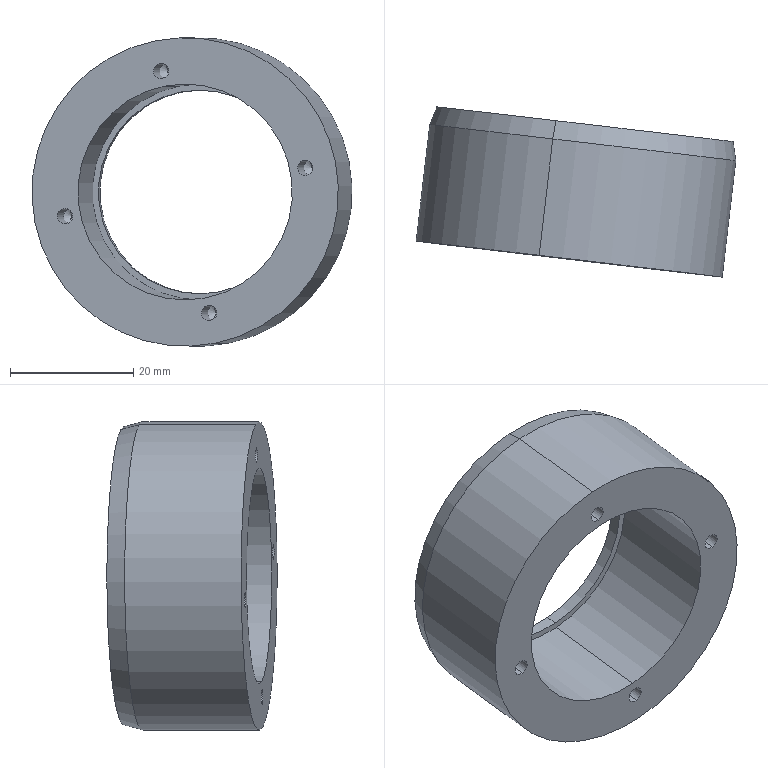Component | SolidWorks | 8TC-A17001-91-00UpperAndLowerPressAssembly-1_8TC-A17001-91-04PressureRoller-1 | 1 solid | 27 faces | box 51.88 x 27.59 x 50 mm | volume 21885 mm3 | cylinder 14 | cone 10 | plane 3 | commonest cylinder face diameters 2.5 x8 33 x2 50 x2 35 x2 | material Cr12MoV
STEP:
#1=COLOUR_RGB('',0.7922,0.8196,0.9333);
#2=FILL_AREA_STYLE_COLOUR('',#1);
#3=FILL_AREA_STYLE('',(#2));
#4=SURFACE_STYLE_FILL_AREA(#3);
#5=SURFACE_SIDE_STYLE('',(#4));
#6=SURFACE_STYLE_USAGE(.BOTH.,#5);
#7=PRESENTATION_STYLE_ASSIGNMENT((#6));
#8=CARTESIAN_POINT('',(0.232,-2.897,-2.771));
#9=VERTEX_POINT('',#8);
#10=CARTESIAN_POINT('',(0.2512,-2.899,-2.868));
#11=VERTEX_POINT('',#10);
#12=CARTESIAN_POINT('',(0.2416,-2.898,-2.819));
#13=DIRECTION('',(-0.1167,-0.9932,0.));
#14=DIRECTION('',(0.1946,-0.02286,-0.9806));
#15=AXIS2_PLACEMENT_3D('',#12,#13,#14);
#16=CIRCLE('',#15,0.04921);
#17=EDGE_CURVE('',#9,#11,#16,.T.);
#18=ORIENTED_EDGE('',*,*,#17,.F.);
#19=CARTESIAN_POINT('',(0.193,-3.229,-2.771));
#20=VERTEX_POINT('',#19);
#21=CARTESIAN_POINT('',(0.193,-3.229,-2.771));
#22=DIRECTION('',(-0.1167,-0.9932,0.));
#23=VECTOR('',#22,39.37);
#24=LINE('',#21,#23);
#25=EDGE_CURVE('',#9,#20,#24,.T.);
#26=ORIENTED_EDGE('',*,*,#25,.T.);
#27=CARTESIAN_POINT('',(0.2122,-3.231,-2.868));
#28=VERTEX_POINT('',#27);
#29=CARTESIAN_POINT('',(0.2026,-3.23,-2.819));
#30=DIRECTION('',(-0.1167,-0.9932,0.));
#31=DIRECTION('',(0.1946,-0.02286,-0.9806));
#32=AXIS2_PLACEMENT_3D('',#29,#30,#31);
#33=CIRCLE('',#32,0.04921);
#34=EDGE_CURVE('',#20,#28,#33,.T.);
#35=ORIENTED_EDGE('',*,*,#34,.T.);
#36=CARTESIAN_POINT('',(0.2122,-3.231,-2.868));
#37=DIRECTION('',(-0.1167,-0.9932,0.));
#38=VECTOR('',#37,39.37);
#39=LINE('',#36,#38);
#40=EDGE_CURVE('',#11,#28,#39,.T.);
#41=ORIENTED_EDGE('',*,*,#40,.F.);
#42=EDGE_LOOP('',(#18,#26,#35,#41));
#43=FACE_OUTER_BOUND('',#42,.T.);
#44=CARTESIAN_POINT('',(0.2026,-3.23,-2.819));
#45=DIRECTION('',(-0.1167,-0.9932,0.));
#46=DIRECTION('',(0.1946,-0.02286,-0.9806));
#47=AXIS2_PLACEMENT_3D('',#44,#45,#46);
#48=CYLINDRICAL_SURFACE('',#47,0.04921);
#49=ADVANCED_FACE('',(#43),#48,.F.);
#50=CARTESIAN_POINT('',(0.2451,-2.868,-2.819));
#51=VERTEX_POINT('',#50);
#52=CARTESIAN_POINT('',(0.2512,-2.899,-2.868));
#53=DIRECTION('',(0.1067,-0.5311,-0.8406));
#54=VECTOR('',#53,39.37);
#55=LINE('',#52,#54);
#56=EDGE_CURVE('',#51,#11,#55,.T.);
#57=ORIENTED_EDGE('',*,*,#56,.F.);
#58=CARTESIAN_POINT('',(0.232,-2.897,-2.771));
#59=DIRECTION('',(-0.2269,-0.4919,0.8406));
#60=VECTOR('',#59,39.37);
#61=LINE('',#58,#60);
#62=EDGE_CURVE('',#51,#9,#61,.T.);
#63=ORIENTED_EDGE('',*,*,#62,.T.);
#64=ORIENTED_EDGE('',*,*,#17,.T.);
#65=EDGE_LOOP('',(#57,#63,#64));
#66=FACE_OUTER_BOUND('',#65,.T.);
#67=CARTESIAN_POINT('',(0.2416,-2.898,-2.819));
#68=DIRECTION('',(-0.1167,-0.9932,0.));
#69=DIRECTION('',(0.1946,-0.02286,-0.9806));
#70=AXIS2_PLACEMENT_3D('',#67,#68,#69);
#71=CONICAL_SURFACE('',#70,0.04921,1.03);
#72=ADVANCED_FACE('',(#66),#71,.F.);
#73=CARTESIAN_POINT('',(0.8457,-2.969,-1.845));
#74=VERTEX_POINT('',#73);
#75=CARTESIAN_POINT('',(0.8648,-2.971,-1.941));
#76=VERTEX_POINT('',#75);
#77=CARTESIAN_POINT('',(0.8553,-2.97,-1.893));
#78=DIRECTION('',(-0.1167,-0.9932,0.));
#79=DIRECTION('',(0.1946,-0.02286,-0.9806));
#80=AXIS2_PLACEMENT_3D('',#77,#78,#79);
#81=CIRCLE('',#80,0.04921);
#82=EDGE_CURVE('',#74,#76,#81,.T.);
#83=ORIENTED_EDGE('',*,*,#82,.F.);
#84=CARTESIAN_POINT('',(0.8066,-3.301,-1.845));
#85=VERTEX_POINT('',#84);
#86=CARTESIAN_POINT('',(0.8066,-3.301,-1.845));
#87=DIRECTION('',(-0.1167,-0.9932,0.));
#88=VECTOR('',#87,39.37);
#89=LINE('',#86,#88);
#90=EDGE_CURVE('',#74,#85,#89,.T.);
#91=ORIENTED_EDGE('',*,*,#90,.T.);
#92=CARTESIAN_POINT('',(0.8258,-3.303,-1.941));
#93=VERTEX_POINT('',#92);
#94=CARTESIAN_POINT('',(0.8162,-3.302,-1.893));
#95=DIRECTION('',(-0.1167,-0.9932,0.));
#96=DIRECTION('',(0.1946,-0.02286,-0.9806));
#97=AXIS2_PLACEMENT_3D('',#94,#95,#96);
#98=CIRCLE('',#97,0.04921);
#99=EDGE_CURVE('',#85,#93,#98,.T.);
#100=ORIENTED_EDGE('',*,*,#99,.T.);
#101=CARTESIAN_POINT('',(0.8258,-3.303,-1.941));
#102=DIRECTION('',(-0.1167,-0.9932,0.));
#103=VECTOR('',#102,39.37);
#104=LINE('',#101,#103);
#105=EDGE_CURVE('',#76,#93,#104,.T.);
#106=ORIENTED_EDGE('',*,*,#105,.F.);
#107=EDGE_LOOP('',(#83,#91,#100,#106));
#108=FACE_OUTER_BOUND('',#107,.T.);
#109=CARTESIAN_POINT('',(0.8162,-3.302,-1.893));
#110=DIRECTION('',(-0.1167,-0.9932,0.));
#111=DIRECTION('',(0.1946,-0.02286,-0.9806));
#112=AXIS2_PLACEMENT_3D('',#109,#110,#111);
#113=CYLINDRICAL_SURFACE('',#112,0.04921);
#114=ADVANCED_FACE('',(#108),#113,.F.);
#115=CARTESIAN_POINT('',(0.8587,-2.94,-1.893));
#116=VERTEX_POINT('',#115);
#117=CARTESIAN_POINT('',(0.8648,-2.971,-1.941));
#118=DIRECTION('',(0.1067,-0.5311,-0.8406));
#119=VECTOR('',#118,39.37);
#120=LINE('',#117,#119);
#121=EDGE_CURVE('',#116,#76,#120,.T.);
#122=ORIENTED_EDGE('',*,*,#121,.F.);
#123=CARTESIAN_POINT('',(0.8457,-2.969,-1.845));
#124=DIRECTION('',(-0.2269,-0.4919,0.8406));
#125=VECTOR('',#124,39.37);
#126=LINE('',#123,#125);
#127=EDGE_CURVE('',#116,#74,#126,.T.);
#128=ORIENTED_EDGE('',*,*,#127,.T.);
#129=ORIENTED_EDGE('',*,*,#82,.T.);
#130=EDGE_LOOP('',(#122,#128,#129));
#131=FACE_OUTER_BOUND('',#130,.T.);
#132=CARTESIAN_POINT('',(0.8553,-2.97,-1.893));
#133=DIRECTION('',(-0.1167,-0.9932,0.));
#134=DIRECTION('',(0.1946,-0.02286,-0.9806));
#135=AXIS2_PLACEMENT_3D('',#132,#133,#134);
#136=CONICAL_SURFACE('',#135,0.04921,1.03);
#137=ADVANCED_FACE('',(#131),#136,.F.);
#138=CARTESIAN_POINT('',(-0.07442,-2.861,-1.227));
#139=VERTEX_POINT('',#138);
#140=CARTESIAN_POINT('',(-0.05527,-2.863,-1.323));
#141=VERTEX_POINT('',#140);
#142=CARTESIAN_POINT('',(-0.06484,-2.862,-1.275));
#143=DIRECTION('',(-0.1167,-0.9932,0.));
#144=DIRECTION('',(0.1946,-0.02286,-0.9806));
#145=AXIS2_PLACEMENT_3D('',#142,#143,#144);
#146=CIRCLE('',#145,0.04921);
#147=EDGE_CURVE('',#139,#141,#146,.T.);
#148=ORIENTED_EDGE('',*,*,#147,.F.);
#149=CARTESIAN_POINT('',(-0.1135,-3.193,-1.227));
#150=VERTEX_POINT('',#149);
#151=CARTESIAN_POINT('',(-0.1135,-3.193,-1.227));
#152=DIRECTION('',(-0.1167,-0.9932,0.));
#153=VECTOR('',#152,39.37);
#154=LINE('',#151,#153);
#155=EDGE_CURVE('',#139,#150,#154,.T.);
#156=ORIENTED_EDGE('',*,*,#155,.T.);
#157=CARTESIAN_POINT('',(-0.09431,-3.195,-1.323));
#158=VERTEX_POINT('',#157);
#159=CARTESIAN_POINT('',(-0.1039,-3.194,-1.275));
#160=DIRECTION('',(-0.1167,-0.9932,0.));
#161=DIRECTION('',(0.1946,-0.02286,-0.9806));
#162=AXIS2_PLACEMENT_3D('',#159,#160,#161);
#163=CIRCLE('',#162,0.04921);
#164=EDGE_CURVE('',#150,#158,#163,.T.);
#165=ORIENTED_EDGE('',*,*,#164,.T.);
#166=CARTESIAN_POINT('',(-0.09431,-3.195,-1.323));
#167=DIRECTION('',(-0.1167,-0.9932,0.));
#168=VECTOR('',#167,39.37);
#169=LINE('',#166,#168);
#170=EDGE_CURVE('',#141,#158,#169,.T.);
#171=ORIENTED_EDGE('',*,*,#170,.F.);
#172=EDGE_LOOP('',(#148,#156,#165,#171));
#173=FACE_OUTER_BOUND('',#172,.T.);
#174=CARTESIAN_POINT('',(-0.1039,-3.194,-1.275));
#175=DIRECTION('',(-0.1167,-0.9932,0.));
#176=DIRECTION('',(0.1946,-0.02286,-0.9806));
#177=AXIS2_PLACEMENT_3D('',#174,#175,#176);
#178=CYLINDRICAL_SURFACE('',#177,0.04921);
#179=ADVANCED_FACE('',(#173),#178,.F.);
#180=CARTESIAN_POINT('',(-0.0614,-2.832,-1.275));
#181=VERTEX_POINT('',#180);
#182=CARTESIAN_POINT('',(-0.05527,-2.863,-1.323));
#183=DIRECTION('',(0.1067,-0.5311,-0.8406));
#184=VECTOR('',#183,39.37);
#185=LINE('',#182,#184);
#186=EDGE_CURVE('',#181,#141,#185,.T.);
#187=ORIENTED_EDGE('',*,*,#186,.F.);
#188=CARTESIAN_POINT('',(-0.07442,-2.861,-1.227));
#189=DIRECTION('',(-0.2269,-0.4919,0.8406));
#190=VECTOR('',#189,39.37);
#191=LINE('',#188,#190);
#192=EDGE_CURVE('',#181,#139,#191,.T.);
#193=ORIENTED_EDGE('',*,*,#192,.T.);
#194=ORIENTED_EDGE('',*,*,#147,.T.);
#195=EDGE_LOOP('',(#187,#193,#194));
#196=FACE_OUTER_BOUND('',#195,.T.);
#197=CARTESIAN_POINT('',(-0.06484,-2.862,-1.275));
#198=DIRECTION('',(-0.1167,-0.9932,0.));
#199=DIRECTION('',(0.1946,-0.02286,-0.9806));
#200=AXIS2_PLACEMENT_3D('',#197,#198,#199);
#201=CONICAL_SURFACE('',#200,0.04921,1.03);
#202=ADVANCED_FACE('',(#196),#201,.F.);
#203=CARTESIAN_POINT('',(-0.6881,-2.788,-2.153));
#204=VERTEX_POINT('',#203);
#205=CARTESIAN_POINT('',(-0.6689,-2.791,-2.25));
#206=VERTEX_POINT('',#205);
#207=CARTESIAN_POINT('',(-0.6785,-2.79,-2.202));
#208=DIRECTION('',(-0.1167,-0.9932,0.));
#209=DIRECTION('',(0.1946,-0.02286,-0.9806));
#210=AXIS2_PLACEMENT_3D('',#207,#208,#209);
#211=CIRCLE('',#210,0.04921);
#212=EDGE_CURVE('',#204,#206,#211,.T.);
#213=ORIENTED_EDGE('',*,*,#212,.F.);
#214=CARTESIAN_POINT('',(-0.7271,-3.121,-2.153));
#215=VERTEX_POINT('',#214);
#216=CARTESIAN_POINT('',(-0.7271,-3.121,-2.153));
#217=DIRECTION('',(-0.1167,-0.9932,0.));
#218=VECTOR('',#217,39.37);
#219=LINE('',#216,#218);
#220=EDGE_CURVE('',#204,#215,#219,.T.);
#221=ORIENTED_EDGE('',*,*,#220,.T.);
#222=CARTESIAN_POINT('',(-0.7079,-3.123,-2.25));
#223=VERTEX_POINT('',#222);
#224=CARTESIAN_POINT('',(-0.7175,-3.122,-2.202));
#225=DIRECTION('',(-0.1167,-0.9932,0.));
#226=DIRECTION('',(0.1946,-0.02286,-0.9806));
#227=AXIS2_PLACEMENT_3D('',#224,#225,#226);
#228=CIRCLE('',#227,0.04921);
#229=EDGE_CURVE('',#215,#223,#228,.T.);
#230=ORIENTED_EDGE('',*,*,#229,.T.);
#231=CARTESIAN_POINT('',(-0.7079,-3.123,-2.25));
#232=DIRECTION('',(-0.1167,-0.9932,0.));
#233=VECTOR('',#232,39.37);
#234=LINE('',#231,#233);
#235=EDGE_CURVE('',#206,#223,#234,.T.);
#236=ORIENTED_EDGE('',*,*,#235,.F.);
#237=EDGE_LOOP('',(#213,#221,#230,#236));
#238=FACE_OUTER_BOUND('',#237,.T.);
#239=CARTESIAN_POINT('',(-0.7175,-3.122,-2.202));
#240=DIRECTION('',(-0.1167,-0.9932,0.));
#241=DIRECTION('',(0.1946,-0.02286,-0.9806));
#242=AXIS2_PLACEMENT_3D('',#239,#240,#241);
#243=CYLINDRICAL_SURFACE('',#242,0.04921);
#244=ADVANCED_FACE('',(#238),#243,.F.);
#245=CARTESIAN_POINT('',(-0.675,-2.76,-2.202));
#246=VERTEX_POINT('',#245);
#247=CARTESIAN_POINT('',(-0.6689,-2.791,-2.25));
#248=DIRECTION('',(0.1067,-0.5311,-0.8406));
#249=VECTOR('',#248,39.37);
#250=LINE('',#247,#249);
#251=EDGE_CURVE('',#246,#206,#250,.T.);
#252=ORIENTED_EDGE('',*,*,#251,.F.);
#253=CARTESIAN_POINT('',(-0.6881,-2.788,-2.153));
#254=DIRECTION('',(-0.2269,-0.4919,0.8406));
#255=VECTOR('',#254,39.37);
#256=LINE('',#253,#255);
#257=EDGE_CURVE('',#246,#204,#256,.T.);
#258=ORIENTED_EDGE('',*,*,#257,.T.);
#259=ORIENTED_EDGE('',*,*,#212,.T.);
#260=EDGE_LOOP('',(#252,#258,#259));
#261=FACE_OUTER_BOUND('',#260,.T.);
#262=CARTESIAN_POINT('',(-0.6785,-2.79,-2.202));
#263=DIRECTION('',(-0.1167,-0.9932,0.));
#264=DIRECTION('',(0.1946,-0.02286,-0.9806));
#265=AXIS2_PLACEMENT_3D('',#262,#263,#264);
#266=CONICAL_SURFACE('',#265,0.04921,1.03);
#267=ADVANCED_FACE('',(#261),#266,.F.);
#268=CARTESIAN_POINT('',(0.2676,-2.445,-2.684));
#269=VERTEX_POINT('',#268);
#270=CARTESIAN_POINT('',(0.01479,-2.415,-1.41));
#271=VERTEX_POINT('',#270);
#272=CARTESIAN_POINT('',(0.1412,-2.43,-2.047));
#273=DIRECTION('',(0.1167,0.9932,-0.));
#274=DIRECTION('',(-0.1946,0.02286,0.9806));
#275=AXIS2_PLACEMENT_3D('',#272,#273,#274);
#276=CIRCLE('',#275,0.6496);
#277=EDGE_CURVE('',#269,#271,#276,.T.);
#278=ORIENTED_EDGE('',*,*,#277,.F.);
#279=CARTESIAN_POINT('',(0.2768,-2.367,-2.684));
#280=VERTEX_POINT('',#279);
#281=CARTESIAN_POINT('',(0.2676,-2.445,-2.684));
#282=DIRECTION('',(0.1167,0.9932,-0.));
#283=VECTOR('',#282,39.37);
#284=LINE('',#281,#283);
#285=EDGE_CURVE('',#269,#280,#284,.T.);
#286=ORIENTED_EDGE('',*,*,#285,.T.);
#287=CARTESIAN_POINT('',(0.02398,-2.337,-1.41));
#288=VERTEX_POINT('',#287);
#289=CARTESIAN_POINT('',(0.1504,-2.352,-2.047));
#290=DIRECTION('',(0.1167,0.9932,-0.));
#291=DIRECTION('',(-0.1946,0.02286,0.9806));
#292=AXIS2_PLACEMENT_3D('',#289,#290,#291);
#293=CIRCLE('',#292,0.6496);
#294=EDGE_CURVE('',#280,#288,#293,.T.);
#295=ORIENTED_EDGE('',*,*,#294,.T.);
#296=CARTESIAN_POINT('',(0.01479,-2.415,-1.41));
#297=DIRECTION('',(0.1167,0.9932,-0.));
#298=VECTOR('',#297,39.37);
#299=LINE('',#296,#298);
#300=EDGE_CURVE('',#271,#288,#299,.T.);
#301=ORIENTED_EDGE('',*,*,#300,.F.);
#302=EDGE_LOOP('',(#278,#286,#295,#301));
#303=FACE_OUTER_BOUND('',#302,.T.);
#304=CARTESIAN_POINT('',(0.1412,-2.43,-2.047));
#305=DIRECTION('',(0.1167,0.9932,-0.));
#306=DIRECTION('',(-0.1946,0.02286,0.9806));
#307=AXIS2_PLACEMENT_3D('',#304,#305,#306);
#308=CYLINDRICAL_SURFACE('',#307,0.6496);
#309=ADVANCED_FACE('',(#303),#308,.F.);
#310=CARTESIAN_POINT('',(-0.03499,-2.33,-1.113));
#311=VERTEX_POINT('',#310);
#312=CARTESIAN_POINT('',(0.3358,-2.374,-2.981));
#313=VERTEX_POINT('',#312);
#314=CARTESIAN_POINT('',(0.1504,-2.352,-2.047));
#315=DIRECTION('',(0.1167,0.9932,-0.));
#316=DIRECTION('',(-0.1946,0.02286,0.9806));
#317=AXIS2_PLACEMENT_3D('',#314,#315,#316);
#318=CIRCLE('',#317,0.9526);
#319=EDGE_CURVE('',#311,#313,#318,.T.);
#320=ORIENTED_EDGE('',*,*,#319,.F.);
#321=CARTESIAN_POINT('',(-0.05493,-2.447,-1.082));
#322=VERTEX_POINT('',#321);
#323=CARTESIAN_POINT('',(-0.05493,-2.447,-1.082));
#324=DIRECTION('',(-0.1631,-0.9534,0.2538));
#325=VECTOR('',#324,39.37);
#326=LINE('',#323,#325);
#327=EDGE_CURVE('',#311,#322,#326,.T.);
#328=ORIENTED_EDGE('',*,*,#327,.T.);
#329=CARTESIAN_POINT('',(0.3282,-2.492,-3.012));
#330=VERTEX_POINT('',#329);
#331=CARTESIAN_POINT('',(0.1366,-2.469,-2.047));
#332=DIRECTION('',(0.1167,0.9932,-0.));
#333=DIRECTION('',(-0.1946,0.02286,0.9806));
#334=AXIS2_PLACEMENT_3D('',#331,#332,#333);
#335=CIRCLE('',#334,0.9843);
#336=EDGE_CURVE('',#322,#330,#335,.T.);
#337=ORIENTED_EDGE('',*,*,#336,.T.);
#338=CARTESIAN_POINT('',(0.3282,-2.492,-3.012));
#339=DIRECTION('',(-0.06232,-0.9652,-0.2538));
#340=VECTOR('',#339,39.37);
#341=LINE('',#338,#340);
#342=EDGE_CURVE('',#313,#330,#341,.T.);
#343=ORIENTED_EDGE('',*,*,#342,.F.);
#344=EDGE_LOOP('',(#320,#328,#337,#343));
#345=FACE_OUTER_BOUND('',#344,.T.);
#346=CARTESIAN_POINT('',(0.1366,-2.469,-2.047));
#347=DIRECTION('',(-0.1167,-0.9932,0.));
#348=DIRECTION('',(0.1946,-0.02286,-0.9806));
#349=AXIS2_PLACEMENT_3D('',#346,#347,#348);
#350=CONICAL_SURFACE('',#349,0.9843,0.2618);
#351=ADVANCED_FACE('',(#345),#350,.T.);
#352=ORIENTED_EDGE('',*,*,#336,.F.);
#353=CARTESIAN_POINT('',(-0.1422,-3.19,-1.082));
#354=VERTEX_POINT('',#353);
#355=CARTESIAN_POINT('',(-0.04115,-2.329,-1.082));
#356=DIRECTION('',(-0.1167,-0.9932,0.));
#357=VECTOR('',#356,39.37);
#358=LINE('',#355,#357);
#359=EDGE_CURVE('',#322,#354,#358,.T.);
#360=ORIENTED_EDGE('',*,*,#359,.T.);
#361=CARTESIAN_POINT('',(0.2409,-3.235,-3.012));
#362=VERTEX_POINT('',#361);
#363=CARTESIAN_POINT('',(0.04935,-3.212,-2.047));
#364=DIRECTION('',(0.1167,0.9932,-0.));
#365=DIRECTION('',(-0.1946,0.02286,0.9806));
#366=AXIS2_PLACEMENT_3D('',#363,#364,#365);
#367=CIRCLE('',#366,0.9843);
#368=EDGE_CURVE('',#354,#362,#367,.T.);
#369=ORIENTED_EDGE('',*,*,#368,.T.);
#370=CARTESIAN_POINT('',(0.3419,-2.374,-3.012));
#371=DIRECTION('',(-0.1167,-0.9932,0.));
#372=VECTOR('',#371,39.37);
#373=LINE('',#370,#372);
#374=EDGE_CURVE('',#330,#362,#373,.T.);
#375=ORIENTED_EDGE('',*,*,#374,.F.);
#376=EDGE_LOOP('',(#352,#360,#369,#375));
#377=FACE_OUTER_BOUND('',#376,.T.);
#378=CARTESIAN_POINT('',(0.1504,-2.352,-2.047));
#379=DIRECTION('',(-0.1167,-0.9932,0.));
#380=DIRECTION('',(0.1946,-0.02286,-0.9806));
#381=AXIS2_PLACEMENT_3D('',#378,#379,#380);
#382=CYLINDRICAL_SURFACE('',#381,0.9843);
#383=ADVANCED_FACE('',(#377),#382,.T.);
#384=CARTESIAN_POINT('',(0.2753,-2.446,-2.723));
#385=VERTEX_POINT('',#384);
#386=CARTESIAN_POINT('',(0.007131,-2.414,-1.372));
#387=VERTEX_POINT('',#386);
#388=CARTESIAN_POINT('',(0.1412,-2.43,-2.047));
#389=DIRECTION('',(0.1167,0.9932,-0.));
#390=DIRECTION('',(-0.1946,0.02286,0.9806));
#391=AXIS2_PLACEMENT_3D('',#388,#389,#390);
#392=CIRCLE('',#391,0.689);
#393=EDGE_CURVE('',#385,#387,#392,.T.);
#394=ORIENTED_EDGE('',*,*,#393,.T.);
#395=CARTESIAN_POINT('',(-0.08473,-3.196,-1.372));
#396=VERTEX_POINT('',#395);
#397=CARTESIAN_POINT('',(0.01632,-2.336,-1.372));
#398=DIRECTION('',(-0.1167,-0.9932,0.));
#399=VECTOR('',#398,39.37);
#400=LINE('',#397,#399);
#401=EDGE_CURVE('',#387,#396,#400,.T.);
#402=ORIENTED_EDGE('',*,*,#401,.T.);
#403=CARTESIAN_POINT('',(0.1834,-3.228,-2.723));
#404=VERTEX_POINT('',#403);
#405=CARTESIAN_POINT('',(0.04935,-3.212,-2.047));
#406=DIRECTION('',(0.1167,0.9932,-0.));
#407=DIRECTION('',(-0.1946,0.02286,0.9806));
#408=AXIS2_PLACEMENT_3D('',#405,#406,#407);
#409=CIRCLE('',#408,0.689);
#410=EDGE_CURVE('',#404,#396,#409,.T.);
#411=ORIENTED_EDGE('',*,*,#410,.F.);
#412=CARTESIAN_POINT('',(0.2845,-2.368,-2.723));
#413=DIRECTION('',(-0.1167,-0.9932,0.));
#414=VECTOR('',#413,39.37);
#415=LINE('',#412,#414);
#416=EDGE_CURVE('',#385,#404,#415,.T.);
#417=ORIENTED_EDGE('',*,*,#416,.F.);
#418=EDGE_LOOP('',(#394,#402,#411,#417));
#419=FACE_OUTER_BOUND('',#418,.T.);
#420=CARTESIAN_POINT('',(0.1504,-2.352,-2.047));
#421=DIRECTION('',(-0.1167,-0.9932,0.));
#422=DIRECTION('',(0.1946,-0.02286,-0.9806));
#423=AXIS2_PLACEMENT_3D('',#420,#421,#422);
#424=CYLINDRICAL_SURFACE('',#423,0.689);
#425=ADVANCED_FACE('',(#419),#424,.F.);
#426=ORIENTED_EDGE('',*,*,#401,.F.);
#427=CARTESIAN_POINT('',(0.1412,-2.43,-2.047));
#428=DIRECTION('',(0.1167,0.9932,-0.));
#429=DIRECTION('',(-0.1946,0.02286,0.9806));
#430=AXIS2_PLACEMENT_3D('',#427,#428,#429);
#431=CIRCLE('',#430,0.689);
#432=EDGE_CURVE('',#387,#385,#431,.T.);
#433=ORIENTED_EDGE('',*,*,#432,.T.);
#434=ORIENTED_EDGE('',*,*,#416,.T.);
#435=CARTESIAN_POINT('',(0.04935,-3.212,-2.047));
#436=DIRECTION('',(0.1167,0.9932,-0.));
#437=DIRECTION('',(-0.1946,0.02286,0.9806));
#438=AXIS2_PLACEMENT_3D('',#435,#436,#437);
#439=CIRCLE('',#438,0.689);
#440=EDGE_CURVE('',#396,#404,#439,.T.);
#441=ORIENTED_EDGE('',*,*,#440,.F.);
#442=EDGE_LOOP('',(#426,#433,#434,#441));
#443=FACE_OUTER_BOUND('',#442,.T.);
#444=CARTESIAN_POINT('',(0.1504,-2.352,-2.047));
#445=DIRECTION('',(-0.1167,-0.9932,0.));
#446=DIRECTION('',(0.1946,-0.02286,-0.9806));
#447=AXIS2_PLACEMENT_3D('',#444,#445,#446);
#448=CYLINDRICAL_SURFACE('',#447,0.689);
#449=ADVANCED_FACE('',(#443),#448,.F.);
#450=CARTESIAN_POINT('',(0.1504,-2.352,-2.047));
#451=DIRECTION('',(0.1167,0.9932,-0.));
#452=DIRECTION('',(-0.1946,0.02286,0.9806));
#453=AXIS2_PLACEMENT_3D('',#450,#451,#452);
#454=CIRCLE('',#453,0.9526);
#455=EDGE_CURVE('',#313,#311,#454,.T.);
#456=ORIENTED_EDGE('',*,*,#455,.T.);
#457=ORIENTED_EDGE('',*,*,#319,.T.);
#458=EDGE_LOOP('',(#456,#457));
#459=FACE_OUTER_BOUND('',#458,.T.);
#460=CARTESIAN_POINT('',(0.1504,-2.352,-2.047));
#461=DIRECTION('',(0.1167,0.9932,-0.));
#462=DIRECTION('',(-0.1946,0.02286,0.9806));
#463=AXIS2_PLACEMENT_3D('',#460,#461,#462);
#464=CIRCLE('',#463,0.6496);
#465=EDGE_CURVE('',#288,#280,#464,.T.);
#466=ORIENTED_EDGE('',*,*,#465,.F.);
#467=ORIENTED_EDGE('',*,*,#294,.F.);
#468=EDGE_LOOP('',(#466,#467));
#469=FACE_BOUND('',#468,.T.);
#470=CARTESIAN_POINT('',(0.1504,-2.352,-2.047));
#471=DIRECTION('',(0.1167,0.9932,-0.));
#472=DIRECTION('',(-0.1946,0.02286,0.9806));
#473=AXIS2_PLACEMENT_3D('',#470,#471,#472);
#474=PLANE('',#473);
#475=ADVANCED_FACE('',(#459,#469),#474,.T.);
#476=CARTESIAN_POINT('',(0.2026,-3.23,-2.819));
#477=DIRECTION('',(-0.1167,-0.9932,0.));
#478=DIRECTION('',(0.1946,-0.02286,-0.9806));
#479=AXIS2_PLACEMENT_3D('',#476,#477,#478);
#480=CIRCLE('',#479,0.04921);
#481=EDGE_CURVE('',#28,#20,#480,.T.);
#482=ORIENTED_EDGE('',*,*,#481,.F.);
#483=ORIENTED_EDGE('',*,*,#34,.F.);
#484=EDGE_LOOP('',(#482,#483));
#485=FACE_BOUND('',#484,.T.);
#486=CARTESIAN_POINT('',(0.8162,-3.302,-1.893));
#487=DIRECTION('',(-0.1167,-0.9932,0.));
#488=DIRECTION('',(0.1946,-0.02286,-0.9806));
#489=AXIS2_PLACEMENT_3D('',#486,#487,#488);
#490=CIRCLE('',#489,0.04921);
#491=EDGE_CURVE('',#93,#85,#490,.T.);
#492=ORIENTED_EDGE('',*,*,#491,.F.);
#493=ORIENTED_EDGE('',*,*,#99,.F.);
#494=EDGE_LOOP('',(#492,#493));
#495=FACE_BOUND('',#494,.T.);
#496=CARTESIAN_POINT('',(-0.1039,-3.194,-1.275));
#497=DIRECTION('',(-0.1167,-0.9932,0.));
#498=DIRECTION('',(0.1946,-0.02286,-0.9806));
#499=AXIS2_PLACEMENT_3D('',#496,#497,#498);
#500=CIRCLE('',#499,0.04921);
#501=EDGE_CURVE('',#158,#150,#500,.T.);
#502=ORIENTED_EDGE('',*,*,#501,.F.);
#503=ORIENTED_EDGE('',*,*,#164,.F.);
#504=EDGE_LOOP('',(#502,#503));
#505=FACE_BOUND('',#504,.T.);
#506=CARTESIAN_POINT('',(-0.7175,-3.122,-2.202));
#507=DIRECTION('',(-0.1167,-0.9932,0.));
#508=DIRECTION('',(0.1946,-0.02286,-0.9806));
#509=AXIS2_PLACEMENT_3D('',#506,#507,#508);
#510=CIRCLE('',#509,0.04921);
#511=EDGE_CURVE('',#223,#215,#510,.T.);
#512=ORIENTED_EDGE('',*,*,#511,.F.);
#513=ORIENTED_EDGE('',*,*,#229,.F.);
#514=EDGE_LOOP('',(#512,#513));
#515=FACE_BOUND('',#514,.T.);
#516=CARTESIAN_POINT('',(0.04935,-3.212,-2.047));
#517=DIRECTION('',(0.1167,0.9932,-0.));
#518=DIRECTION('',(-0.1946,0.02286,0.9806));
#519=AXIS2_PLACEMENT_3D('',#516,#517,#518);
#520=CIRCLE('',#519,0.9843);
#521=EDGE_CURVE('',#362,#354,#520,.T.);
#522=ORIENTED_EDGE('',*,*,#521,.F.);
#523=ORIENTED_EDGE('',*,*,#368,.F.);
#524=EDGE_LOOP('',(#522,#523));
#525=FACE_OUTER_BOUND('',#524,.T.);
#526=ORIENTED_EDGE('',*,*,#410,.T.);
#527=ORIENTED_EDGE('',*,*,#440,.T.);
#528=EDGE_LOOP('',(#526,#527));
#529=FACE_BOUND('',#528,.T.);
#530=CARTESIAN_POINT('',(0.04935,-3.212,-2.047));
#531=DIRECTION('',(0.1167,0.9932,-0.));
#532=DIRECTION('',(-0.1946,0.02286,0.9806));
#533=AXIS2_PLACEMENT_3D('',#530,#531,#532);
#534=PLANE('',#533);
#535=ADVANCED_FACE('',(#485,#495,#505,#515,#525,#529),#534,.F.);
#536=ORIENTED_EDGE('',*,*,#359,.F.);
#537=CARTESIAN_POINT('',(0.1366,-2.469,-2.047));
#538=DIRECTION('',(0.1167,0.9932,-0.));
#539=DIRECTION('',(-0.1946,0.02286,0.9806));
#540=AXIS2_PLACEMENT_3D('',#537,#538,#539);
#541=CIRCLE('',#540,0.9843);
#542=EDGE_CURVE('',#330,#322,#541,.T.);
#543=ORIENTED_EDGE('',*,*,#542,.F.);
#544=ORIENTED_EDGE('',*,*,#374,.T.);
#545=ORIENTED_EDGE('',*,*,#521,.T.);
#546=EDGE_LOOP('',(#536,#543,#544,#545));
#547=FACE_OUTER_BOUND('',#546,.T.);
#548=CARTESIAN_POINT('',(0.1504,-2.352,-2.047));
#549=DIRECTION('',(-0.1167,-0.9932,0.));
#550=DIRECTION('',(0.1946,-0.02286,-0.9806));
#551=AXIS2_PLACEMENT_3D('',#548,#549,#550);
#552=CYLINDRICAL_SURFACE('',#551,0.9843);
#553=ADVANCED_FACE('',(#547),#552,.T.);
#554=ORIENTED_EDGE('',*,*,#327,.F.);
#555=ORIENTED_EDGE('',*,*,#455,.F.);
#556=ORIENTED_EDGE('',*,*,#342,.T.);
#557=ORIENTED_EDGE('',*,*,#542,.T.);
#558=EDGE_LOOP('',(#554,#555,#556,#557));
#559=FACE_OUTER_BOUND('',#558,.T.);
#560=CARTESIAN_POINT('',(0.1366,-2.469,-2.047));
#561=DIRECTION('',(-0.1167,-0.9932,0.));
#562=DIRECTION('',(0.1946,-0.02286,-0.9806));
#563=AXIS2_PLACEMENT_3D('',#560,#561,#562);
#564=CONICAL_SURFACE('',#563,0.9843,0.2618);
#565=ADVANCED_FACE('',(#559),#564,.T.);
#566=CARTESIAN_POINT('',(0.1412,-2.43,-2.047));
#567=DIRECTION('',(0.1167,0.9932,-0.));
#568=DIRECTION('',(-0.1946,0.02286,0.9806));
#569=AXIS2_PLACEMENT_3D('',#566,#567,#568);
#570=CIRCLE('',#569,0.6496);
#571=EDGE_CURVE('',#271,#269,#570,.T.);
#572=ORIENTED_EDGE('',*,*,#571,.T.);
#573=ORIENTED_EDGE('',*,*,#277,.T.);
#574=EDGE_LOOP('',(#572,#573));
#575=FACE_BOUND('',#574,.T.);
#576=ORIENTED_EDGE('',*,*,#393,.F.);
#577=ORIENTED_EDGE('',*,*,#432,.F.);
#578=EDGE_LOOP('',(#576,#577));
#579=FACE_OUTER_BOUND('',#578,.T.);
#580=CARTESIAN_POINT('',(0.1412,-2.43,-2.047));
#581=DIRECTION('',(0.1167,0.9932,-0.));
#582=DIRECTION('',(-0.1946,0.02286,0.9806));
#583=AXIS2_PLACEMENT_3D('',#580,#581,#582);
#584=PLANE('',#583);
#585=ADVANCED_FACE('',(#575,#579),#584,.F.);
#586=ORIENTED_EDGE('',*,*,#285,.F.);
#587=ORIENTED_EDGE('',*,*,#571,.F.);
#588=ORIENTED_EDGE('',*,*,#300,.T.);
#589=ORIENTED_EDGE('',*,*,#465,.T.);
#590=EDGE_LOOP('',(#586,#587,#588,#589));
#591=FACE_OUTER_BOUND('',#590,.T.);
#592=CARTESIAN_POINT('',(0.1412,-2.43,-2.047));
#593=DIRECTION('',(0.1167,0.9932,-0.));
#594=DIRECTION('',(-0.1946,0.02286,0.9806));
#595=AXIS2_PLACEMENT_3D('',#592,#593,#594);
#596=CYLINDRICAL_SURFACE('',#595,0.6496);
#597=ADVANCED_FACE('',(#591),#596,.F.);
#598=ORIENTED_EDGE('',*,*,#257,.F.);
#599=ORIENTED_EDGE('',*,*,#251,.T.);
#600=CARTESIAN_POINT('',(-0.6785,-2.79,-2.202));
#601=DIRECTION('',(-0.1167,-0.9932,0.));
#602=DIRECTION('',(0.1946,-0.02286,-0.9806));
#603=AXIS2_PLACEMENT_3D('',#600,#601,#602);
#604=CIRCLE('',#603,0.04921);
#605=EDGE_CURVE('',#206,#204,#604,.T.);
#606=ORIENTED_EDGE('',*,*,#605,.T.);
#607=EDGE_LOOP('',(#598,#599,#606));
#608=FACE_OUTER_BOUND('',#607,.T.);
#609=CARTESIAN_POINT('',(-0.6785,-2.79,-2.202));
#610=DIRECTION('',(-0.1167,-0.9932,0.));
#611=DIRECTION('',(0.1946,-0.02286,-0.9806));
#612=AXIS2_PLACEMENT_3D('',#609,#610,#611);
#613=CONICAL_SURFACE('',#612,0.04921,1.03);
#614=ADVANCED_FACE('',(#608),#613,.F.);
#615=ORIENTED_EDGE('',*,*,#220,.F.);
#616=ORIENTED_EDGE('',*,*,#605,.F.);
#617=ORIENTED_EDGE('',*,*,#235,.T.);
#618=ORIENTED_EDGE('',*,*,#511,.T.);
#619=EDGE_LOOP('',(#615,#616,#617,#618));
#620=FACE_OUTER_BOUND('',#619,.T.);
#621=CARTESIAN_POINT('',(-0.7175,-3.122,-2.202));
#622=DIRECTION('',(-0.1167,-0.9932,0.));
#623=DIRECTION('',(0.1946,-0.02286,-0.9806));
#624=AXIS2_PLACEMENT_3D('',#621,#622,#623);
#625=CYLINDRICAL_SURFACE('',#624,0.04921);
#626=ADVANCED_FACE('',(#620),#625,.F.);
#627=ORIENTED_EDGE('',*,*,#192,.F.);
#628=ORIENTED_EDGE('',*,*,#186,.T.);
#629=CARTESIAN_POINT('',(-0.06484,-2.862,-1.275));
#630=DIRECTION('',(-0.1167,-0.9932,0.));
#631=DIRECTION('',(0.1946,-0.02286,-0.9806));
#632=AXIS2_PLACEMENT_3D('',#629,#630,#631);
#633=CIRCLE('',#632,0.04921);
#634=EDGE_CURVE('',#141,#139,#633,.T.);
#635=ORIENTED_EDGE('',*,*,#634,.T.);
#636=EDGE_LOOP('',(#627,#628,#635));
#637=FACE_OUTER_BOUND('',#636,.T.);
#638=CARTESIAN_POINT('',(-0.06484,-2.862,-1.275));
#639=DIRECTION('',(-0.1167,-0.9932,0.));
#640=DIRECTION('',(0.1946,-0.02286,-0.9806));
#641=AXIS2_PLACEMENT_3D('',#638,#639,#640);
#642=CONICAL_SURFACE('',#641,0.04921,1.03);
#643=ADVANCED_FACE('',(#637),#642,.F.);
#644=ORIENTED_EDGE('',*,*,#155,.F.);
#645=ORIENTED_EDGE('',*,*,#634,.F.);
#646=ORIENTED_EDGE('',*,*,#170,.T.);
#647=ORIENTED_EDGE('',*,*,#501,.T.);
#648=EDGE_LOOP('',(#644,#645,#646,#647));
#649=FACE_OUTER_BOUND('',#648,.T.);
#650=CARTESIAN_POINT('',(-0.1039,-3.194,-1.275));
#651=DIRECTION('',(-0.1167,-0.9932,0.));
#652=DIRECTION('',(0.1946,-0.02286,-0.9806));
#653=AXIS2_PLACEMENT_3D('',#650,#651,#652);
#654=CYLINDRICAL_SURFACE('',#653,0.04921);
#655=ADVANCED_FACE('',(#649),#654,.F.);
#656=ORIENTED_EDGE('',*,*,#127,.F.);
#657=ORIENTED_EDGE('',*,*,#121,.T.);
#658=CARTESIAN_POINT('',(0.8553,-2.97,-1.893));
#659=DIRECTION('',(-0.1167,-0.9932,0.));
#660=DIRECTION('',(0.1946,-0.02286,-0.9806));
#661=AXIS2_PLACEMENT_3D('',#658,#659,#660);
#662=CIRCLE('',#661,0.04921);
#663=EDGE_CURVE('',#76,#74,#662,.T.);
#664=ORIENTED_EDGE('',*,*,#663,.T.);
#665=EDGE_LOOP('',(#656,#657,#664));
#666=FACE_OUTER_BOUND('',#665,.T.);
#667=CARTESIAN_POINT('',(0.8553,-2.97,-1.893));
#668=DIRECTION('',(-0.1167,-0.9932,0.));
#669=DIRECTION('',(0.1946,-0.02286,-0.9806));
#670=AXIS2_PLACEMENT_3D('',#667,#668,#669);
#671=CONICAL_SURFACE('',#670,0.04921,1.03);
#672=ADVANCED_FACE('',(#666),#671,.F.);
#673=ORIENTED_EDGE('',*,*,#90,.F.);
#674=ORIENTED_EDGE('',*,*,#663,.F.);
#675=ORIENTED_EDGE('',*,*,#105,.T.);
#676=ORIENTED_EDGE('',*,*,#491,.T.);
#677=EDGE_LOOP('',(#673,#674,#675,#676));
#678=FACE_OUTER_BOUND('',#677,.T.);
#679=CARTESIAN_POINT('',(0.8162,-3.302,-1.893));
#680=DIRECTION('',(-0.1167,-0.9932,0.));
#681=DIRECTION('',(0.1946,-0.02286,-0.9806));
#682=AXIS2_PLACEMENT_3D('',#679,#680,#681);
#683=CYLINDRICAL_SURFACE('',#682,0.04921);
#684=ADVANCED_FACE('',(#678),#683,.F.);
#685=ORIENTED_EDGE('',*,*,#62,.F.);
#686=ORIENTED_EDGE('',*,*,#56,.T.);
#687=CARTESIAN_POINT('',(0.2416,-2.898,-2.819));
#688=DIRECTION('',(-0.1167,-0.9932,0.));
#689=DIRECTION('',(0.1946,-0.02286,-0.9806));
#690=AXIS2_PLACEMENT_3D('',#687,#688,#689);
#691=CIRCLE('',#690,0.04921);
#692=EDGE_CURVE('',#11,#9,#691,.T.);
#693=ORIENTED_EDGE('',*,*,#692,.T.);
#694=EDGE_LOOP('',(#685,#686,#693));
#695=FACE_OUTER_BOUND('',#694,.T.);
#696=CARTESIAN_POINT('',(0.2416,-2.898,-2.819));
#697=DIRECTION('',(-0.1167,-0.9932,0.));
#698=DIRECTION('',(0.1946,-0.02286,-0.9806));
#699=AXIS2_PLACEMENT_3D('',#696,#697,#698);
#700=CONICAL_SURFACE('',#699,0.04921,1.03);
#701=ADVANCED_FACE('',(#695),#700,.F.);
#702=ORIENTED_EDGE('',*,*,#25,.F.);
#703=ORIENTED_EDGE('',*,*,#692,.F.);
#704=ORIENTED_EDGE('',*,*,#40,.T.);
#705=ORIENTED_EDGE('',*,*,#481,.T.);
#706=EDGE_LOOP('',(#702,#703,#704,#705));
#707=FACE_OUTER_BOUND('',#706,.T.);
#708=CARTESIAN_POINT('',(0.2026,-3.23,-2.819));
#709=DIRECTION('',(-0.1167,-0.9932,0.));
#710=DIRECTION('',(0.1946,-0.02286,-0.9806));
#711=AXIS2_PLACEMENT_3D('',#708,#709,#710);
#712=CYLINDRICAL_SURFACE('',#711,0.04921);
#713=ADVANCED_FACE('',(#707),#712,.F.);
#714=CLOSED_SHELL('',(#49,#72,#114,#137,#179,#202,#244,#267,#309,#351,#383,#425,#449,#475,#535,#553,#565,#585,#597,#614,#626,#643,#655,#672,#684,#701,#713));
#715=MANIFOLD_SOLID_BREP('',#714);
#716=STYLED_ITEM('',(#7),#715);
#717=PRESENTATION_LAYER_ASSIGNMENT('','',(#716));
#718=(LENGTH_UNIT()NAMED_UNIT(*)SI_UNIT($,.METRE.));
#719=LENGTH_MEASURE_WITH_UNIT(LENGTH_MEASURE(0.0254),#718);
#720=DIMENSIONAL_EXPONENTS(1.,0.,0.,0.,0.,0.,0.);
#721=(CONVERSION_BASED_UNIT('',#719)LENGTH_UNIT()NAMED_UNIT(#720));
#722=UNCERTAINTY_MEASURE_WITH_UNIT(LENGTH_MEASURE(0.00001),#721,'','');
#723=(NAMED_UNIT(*)PLANE_ANGLE_UNIT()SI_UNIT($,.RADIAN.));
#724=(NAMED_UNIT(*)SI_UNIT($,.STERADIAN.)SOLID_ANGLE_UNIT());
#725=(GEOMETRIC_REPRESENTATION_CONTEXT(3)GLOBAL_UNCERTAINTY_ASSIGNED_CONTEXT((#722))GLOBAL_UNIT_ASSIGNED_CONTEXT((#721,#723,#724))REPRESENTATION_CONTEXT('',''));
#726=MECHANICAL_DESIGN_GEOMETRIC_PRESENTATION_REPRESENTATION('',(#716),#725);
#727=CARTESIAN_POINT('',(0.,0.,0.));
#728=DIRECTION('',(0.,0.,1.));
#729=DIRECTION('',(1.,0.,0.));
#730=AXIS2_PLACEMENT_3D('',#727,#728,#729);
#731=(LENGTH_UNIT()NAMED_UNIT(*)SI_UNIT($,.METRE.));
#732=LENGTH_MEASURE_WITH_UNIT(LENGTH_MEASURE(0.0254),#731);
#733=DIMENSIONAL_EXPONENTS(1.,0.,0.,0.,0.,0.,0.);
#734=(CONVERSION_BASED_UNIT('',#732)LENGTH_UNIT()NAMED_UNIT(#733));
#735=UNCERTAINTY_MEASURE_WITH_UNIT(LENGTH_MEASURE(0.00001),#734,'','');
#736=(NAMED_UNIT(*)PLANE_ANGLE_UNIT()SI_UNIT($,.RADIAN.));
#737=(NAMED_UNIT(*)SI_UNIT($,.STERADIAN.)SOLID_ANGLE_UNIT());
#738=(GEOMETRIC_REPRESENTATION_CONTEXT(3)GLOBAL_UNCERTAINTY_ASSIGNED_CONTEXT((#735))GLOBAL_UNIT_ASSIGNED_CONTEXT((#734,#736,#737))REPRESENTATION_CONTEXT('',''));
#739=ADVANCED_BREP_SHAPE_REPRESENTATION('',(#715,#730),#738);